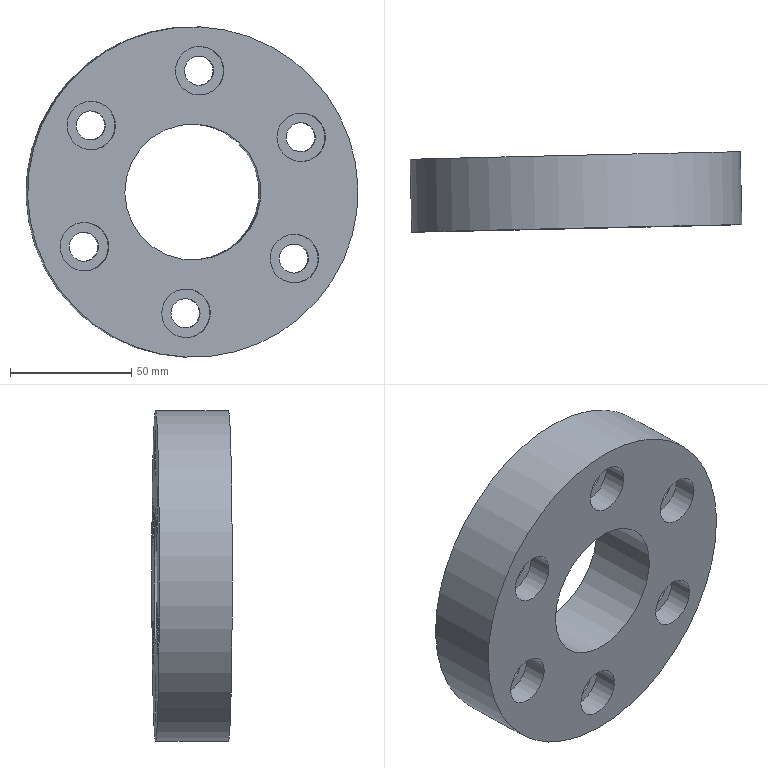Component | NX | 9 | 1 solid | 34 faces | volume 317427 mm3 | cylinder 20 | plane 14 | commonest cylinder face diameters 20 x12 12 x6 136 x1 56 x1